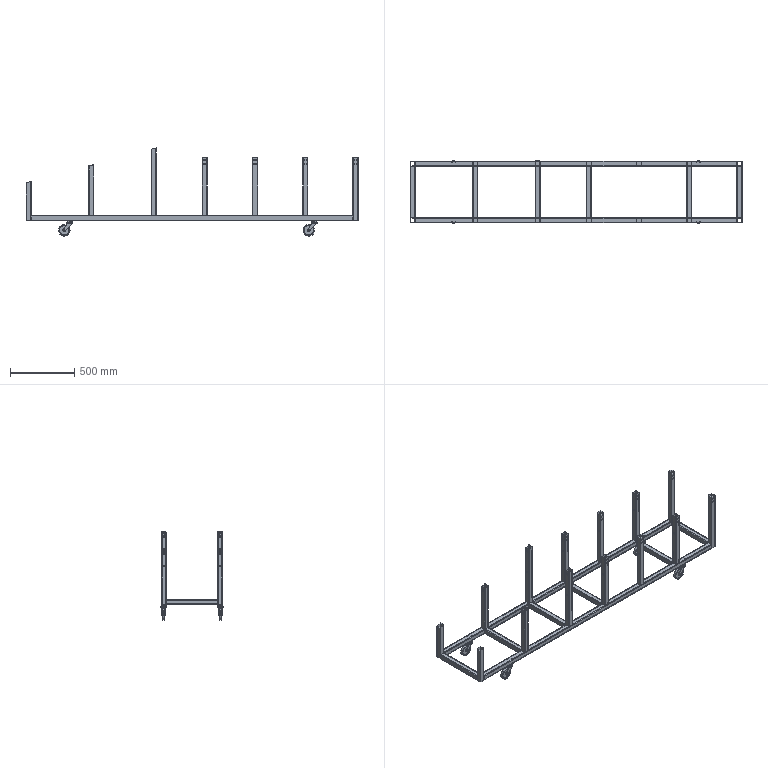Assembly | NX | mm | 34 component files | 42 solids | 840 faces | box 2580 x 490 x 684.65 mm | volume 6733164 mm3 | cylinder 432 | plane 336 | cone 52 | torus 20 | commonest cylinder face diameters 8 x256 6 x52 10 x32 5 x32 16 x16 30 x12 20 x8 75 x8
Bill of materials:
unnamed part 1 | 4 |  | Straight hollow square tube with rounded corners and open ends. It has a cluster of four small through-holes near one end on one face and single holes on the adjacent faces.
unnamed part 2 | 4 |  | Wheel- or pulley-like disc with a raised outer rim, a recessed face and a central hub boss with a small center bore. The hub sticks out on both sides.
unnamed part 3 | 4 |  | Bracket with a circular disc plate and a center hole. Two parallel tapered flat arms hang down from the disc at an angle, and each ends in a rounded lug with a through-hole.
unnamed part 4 | 2 |  | Long, slender hollow square tube with rounded corners and open ends. Small hole clusters sit near each end.
unnamed part 5 | 2 |  | Short hollow square tube with rounded corners. One end is cut at an angle.
unnamed part 6 | 2 |  | Straight hollow square tube with rounded corners and open ends. It has a cluster of four small holes near one end on one face and single holes on the adjacent faces.
unnamed part 7 | 6 |  | Plain straight hollow square tube with rounded corners and square-cut open ends.
unnamed part 8 | 2 |  | Hollow square tube with a fairly thick wall and rounded corners. One end is cut at an angle and there is a single hole on one face.
unnamed part 9 | 2 |  | Hollow square tube with a fairly thick wall and rounded corners. One end is cut at an angle and no holes are visible.
unnamed part 10 | 4 |  | Square flange plate with rounded corners and four corner through-holes. A circular feature sits on the top face. Underneath are a cylindrical body with a rounded bead ring and a small central shaft with a chamfered tip.
unnamed part 11 | 2 |  | Straight hollow square tube with rounded corners and open ends. It has a cluster of four small holes near one end on one face and a single hole near the same end on an adjacent face.
Mates:
1. fix | uni_wheel_base 1 component
2. touch align | uni_wheel_base 1 | uni_wheel_conn_frame 1
3. touch align | uni_wheel_conn_frame 1 | uni_wheel_base 1
4. touch align | uni_wheel_body 1 | uni_wheel_conn_frame 1
5. touch align | uni_wheel_body 1 | uni_wheel_conn_frame 1
6. parallel | uni_wheel_base 1 | uni_wheel_conn_frame 1